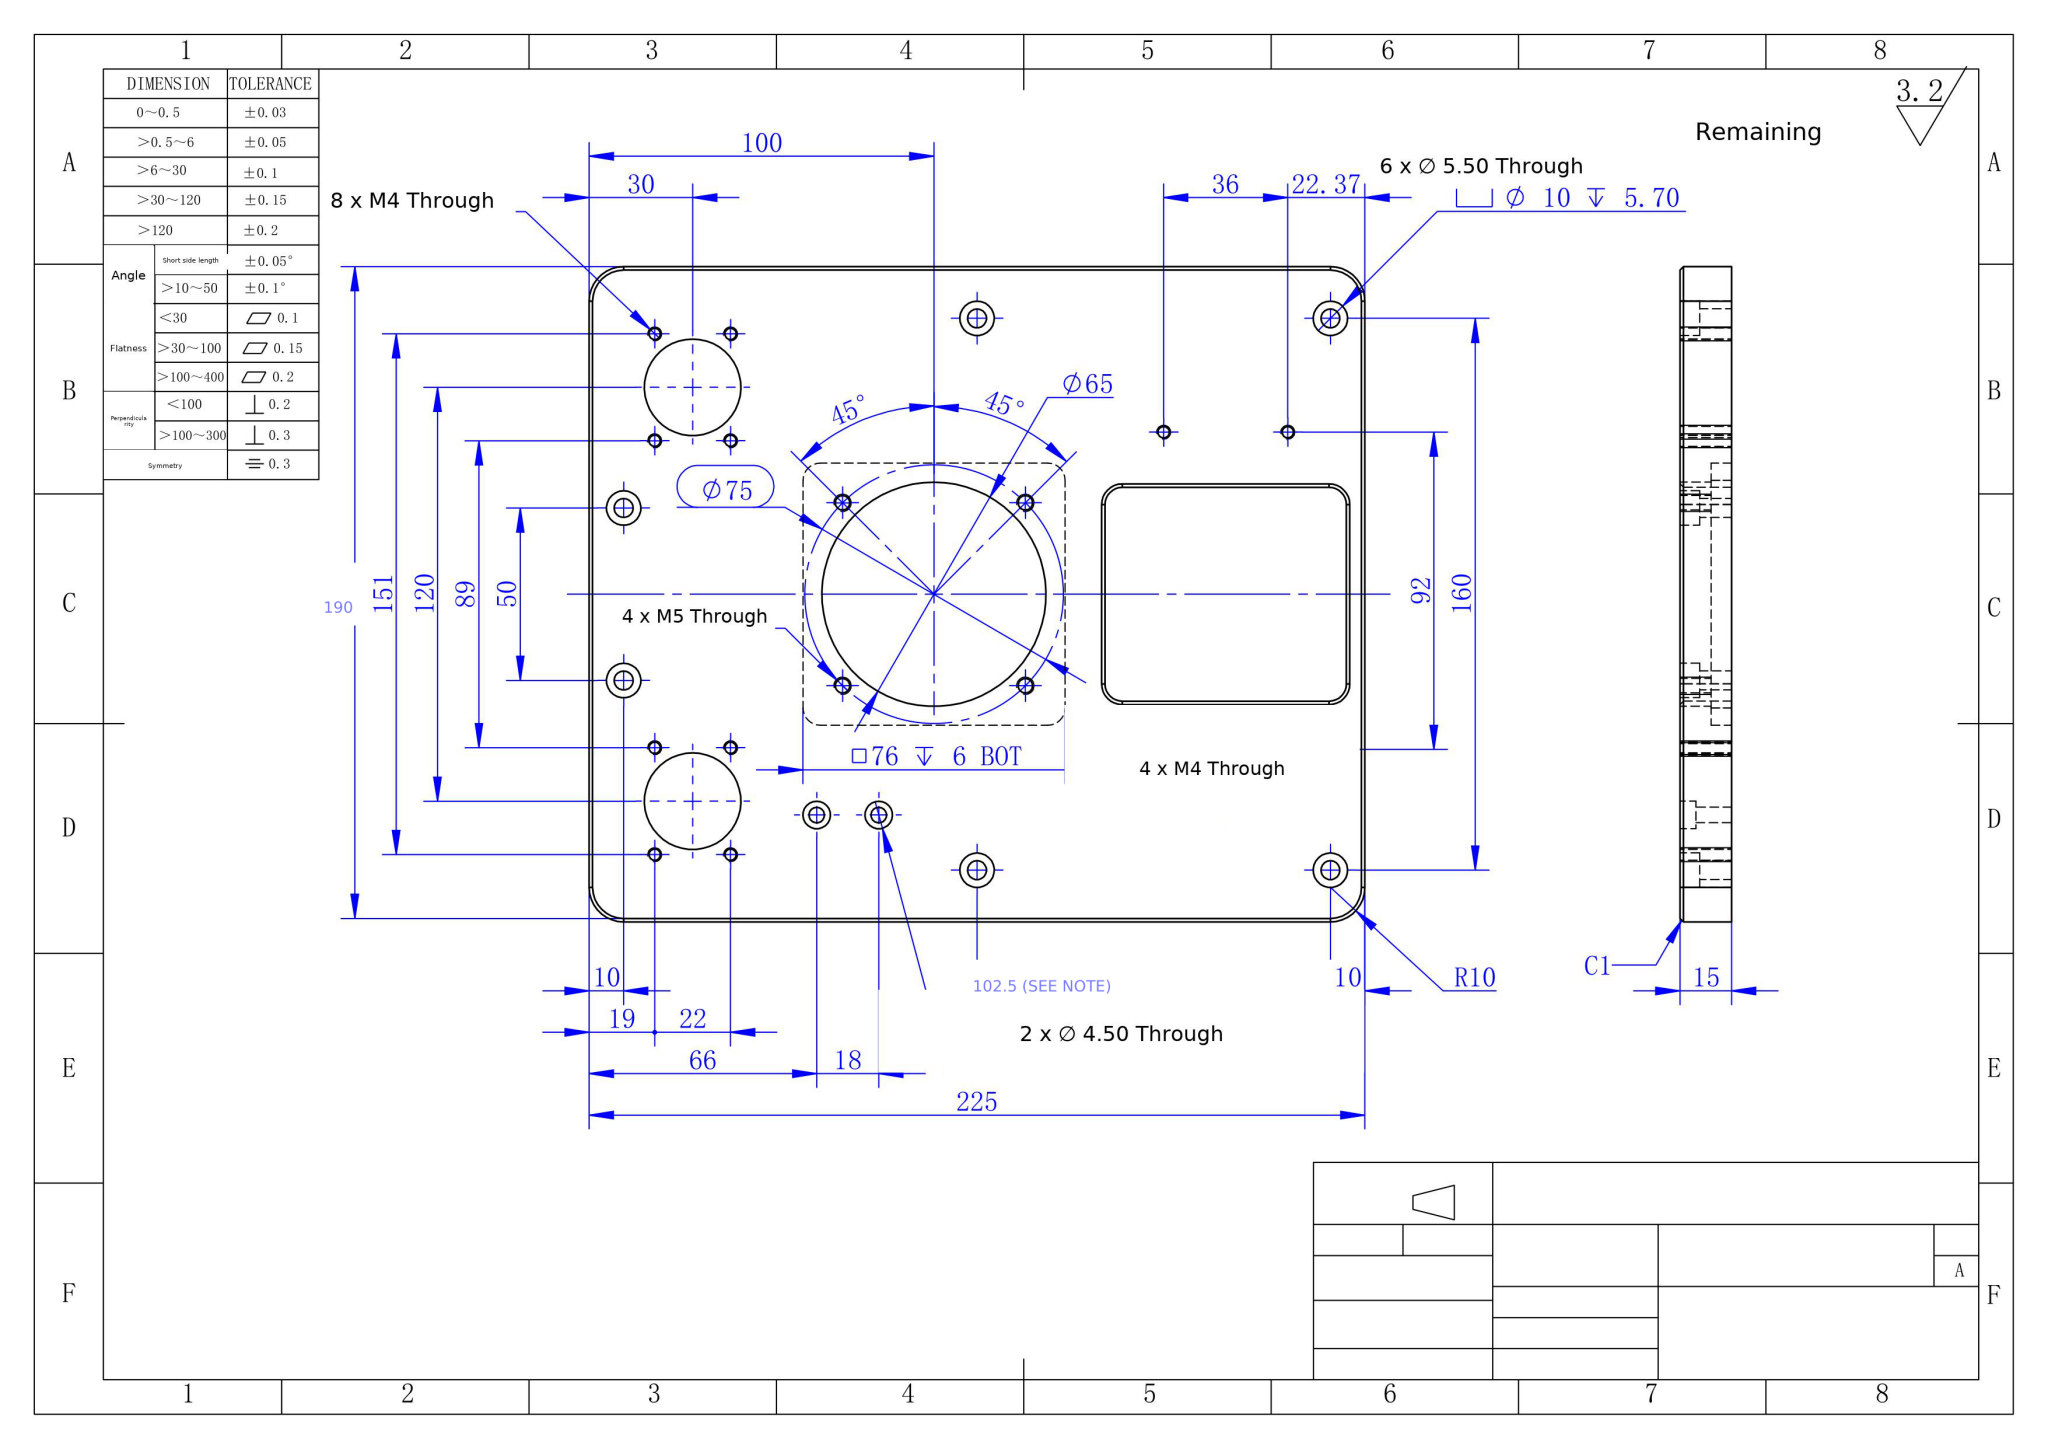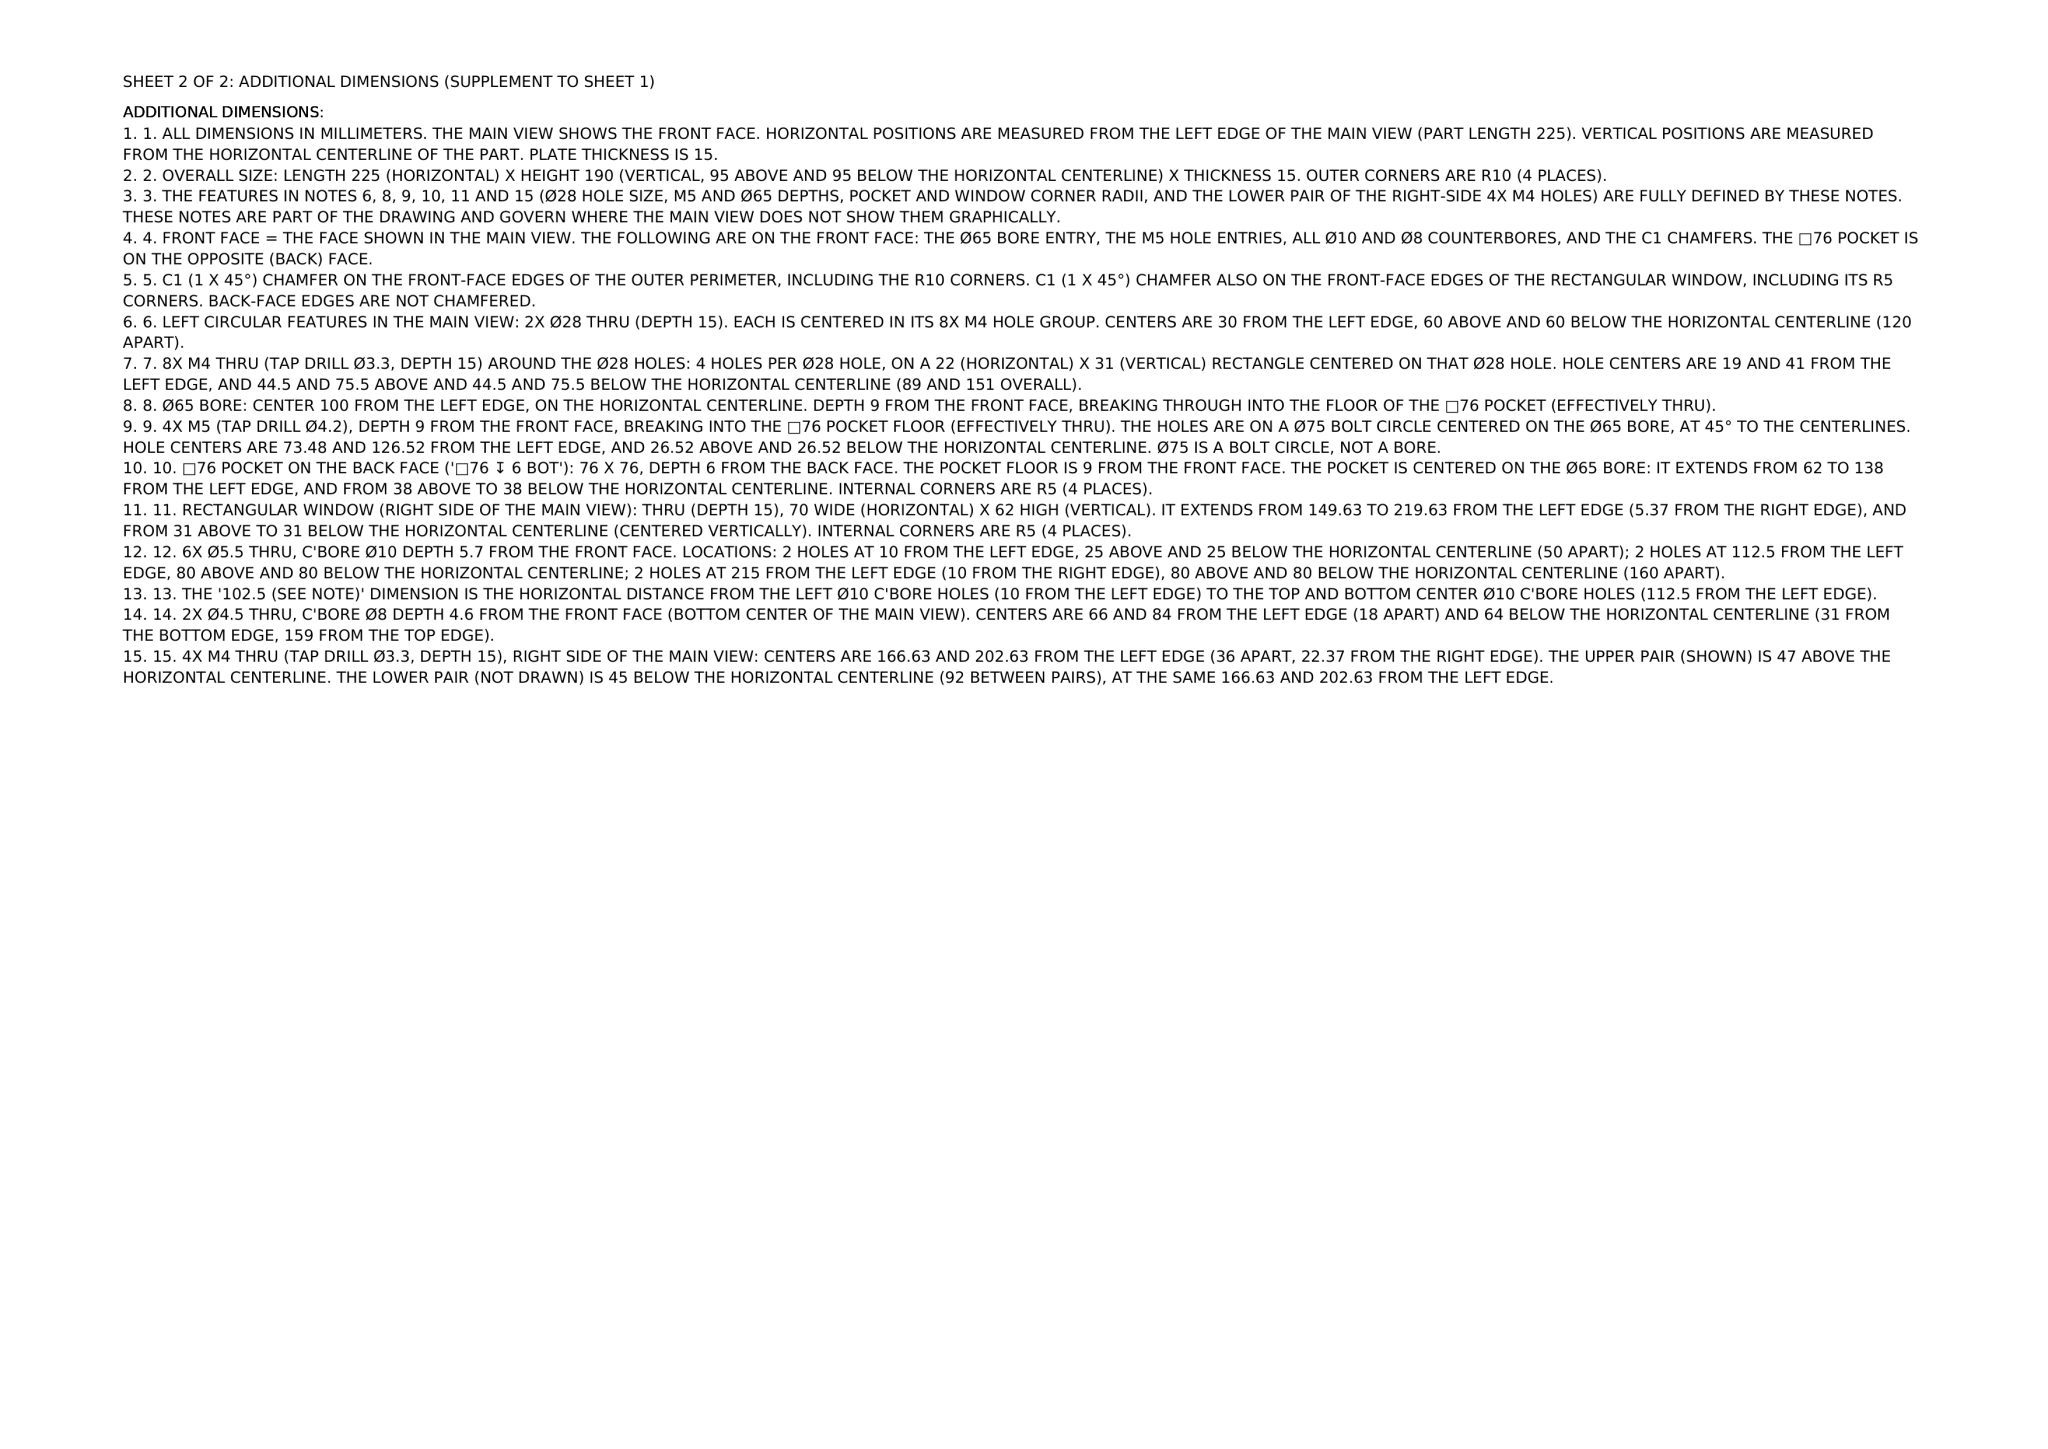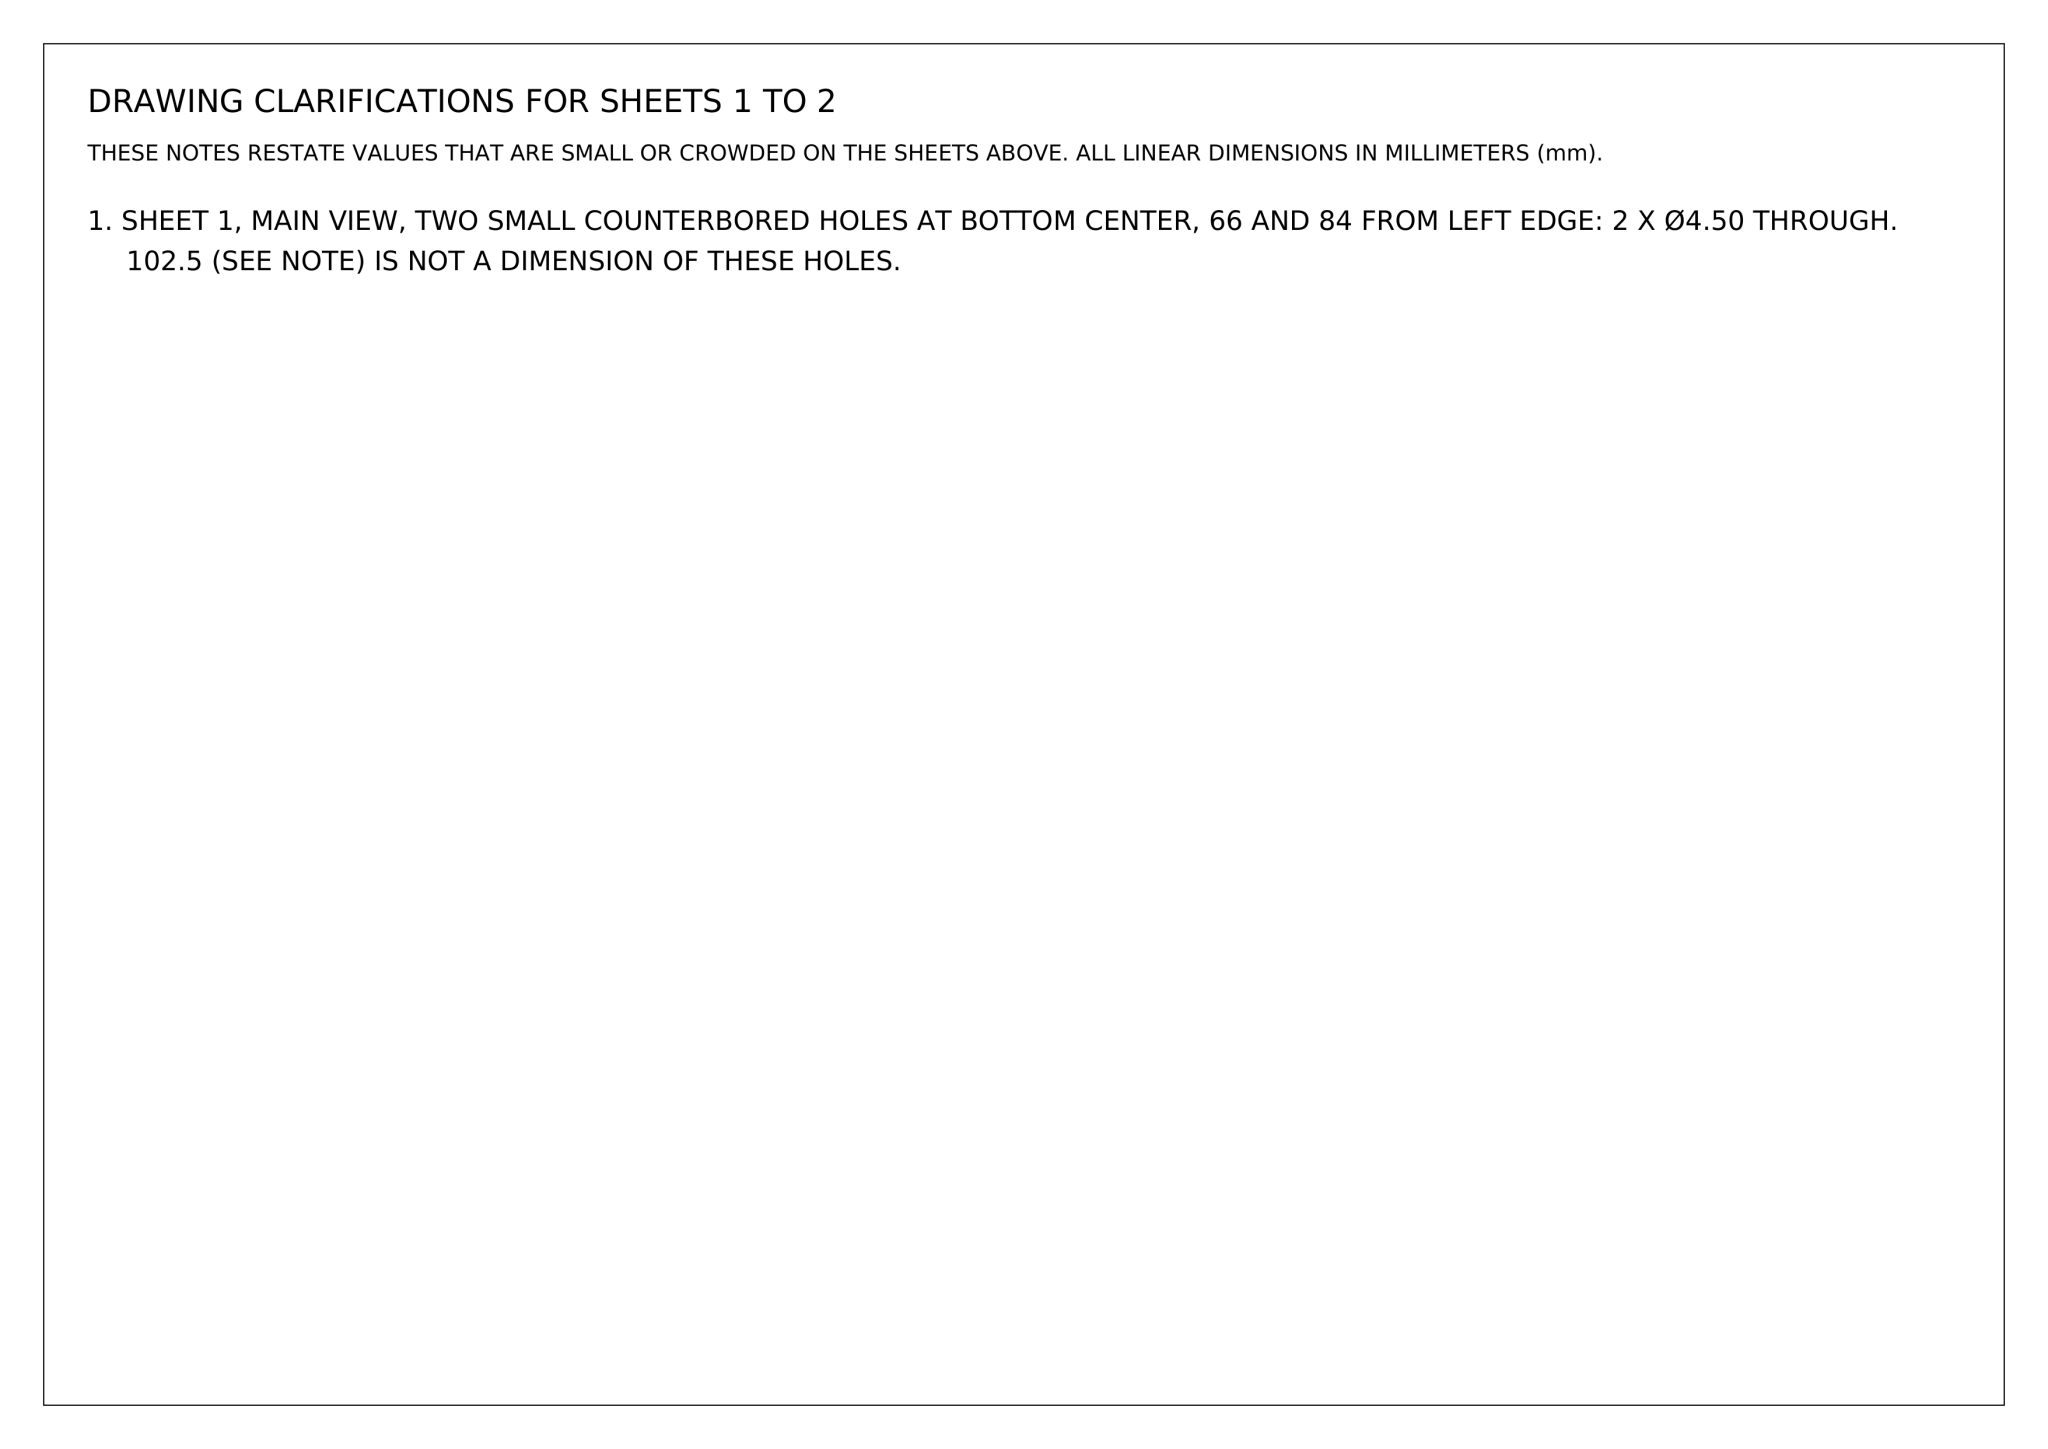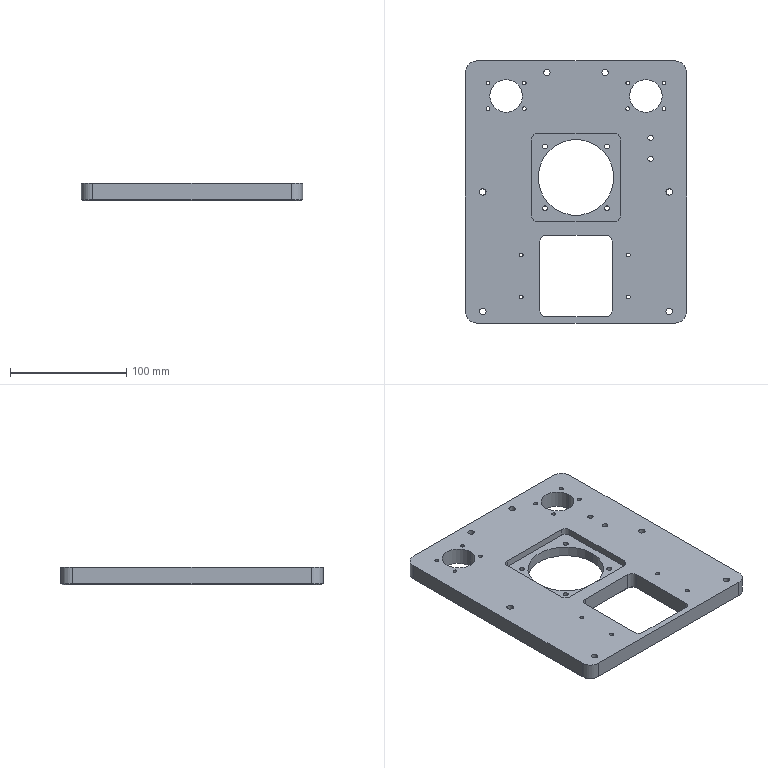Part | NX | mm | 1 solid | 121 faces | box 190 x 225 x 15 mm | volume 484942 mm3 | cylinder 82 | plane 31 | cone 8 | commonest cylinder face diameters 3.3 x24 10 x20 5.5 x12 4.2 x8 8 x4 4.5 x4 28 x4 20 x4